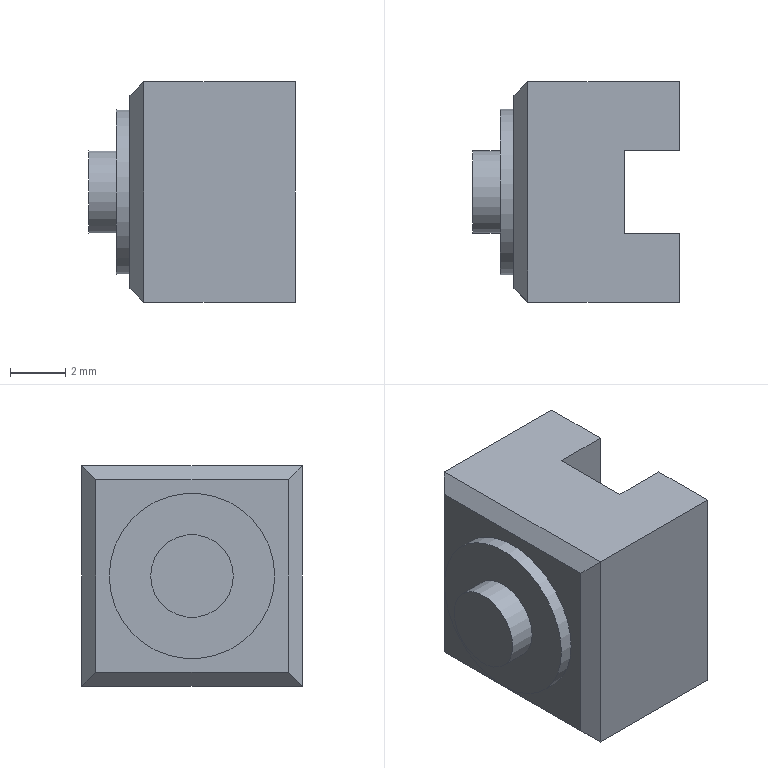Component | NX | IR_THERMAL_IMAGER | 1 solid | 18 faces | box 7.5 x 8 x 8 mm | volume 353 mm3 | plane 16 | cylinder 2 | commonest cylinder face diameters 6 x1 3 x1
STEP:
#1=CARTESIAN_POINT('',(0.,0.,0.));
#2=DIRECTION('',(0.,0.,1.));
#3=DIRECTION('',(1.,0.,0.));
#4=AXIS2_PLACEMENT_3D('',#1,#2,#3);
#5=CARTESIAN_POINT('',(-16.5,4.,12.5));
#6=VERTEX_POINT('',#5);
#7=CARTESIAN_POINT('',(-11.,4.,12.5));
#8=VERTEX_POINT('',#7);
#9=CARTESIAN_POINT('',(-17.,4.,12.5));
#10=DIRECTION('',(1.,0.,0.));
#11=VECTOR('',#10,1.);
#12=LINE('',#9,#11);
#13=CARTESIAN_POINT('',(-17.,4.,12.5));
#14=DIRECTION('',(0.,0.,1.));
#15=DIRECTION('',(0.,1.,-0.));
#16=AXIS2_PLACEMENT_3D('',#13,#14,#15);
#17=PLANE('',#16);
#18=CARTESIAN_POINT('',(0.,0.));
#19=DIRECTION('',(0.,-1.));
#20=VECTOR('',#19,1.);
#21=LINE('',#18,#20);
#22=(GEOMETRIC_REPRESENTATION_CONTEXT(2)PARAMETRIC_REPRESENTATION_CONTEXT()REPRESENTATION_CONTEXT('',''));
#23=DEFINITIONAL_REPRESENTATION('',(#21),#22);
#24=PCURVE('',#17,#23);
#25=CARTESIAN_POINT('',(-17.,4.,4.5));
#26=DIRECTION('',(0.,1.,-0.));
#27=DIRECTION('',(0.,-0.,-1.));
#28=AXIS2_PLACEMENT_3D('',#25,#26,#27);
#29=PLANE('',#28);
#30=CARTESIAN_POINT('',(-8.,0.));
#31=DIRECTION('',(0.,-1.));
#32=VECTOR('',#31,1.);
#33=LINE('',#30,#32);
#34=(GEOMETRIC_REPRESENTATION_CONTEXT(2)PARAMETRIC_REPRESENTATION_CONTEXT()REPRESENTATION_CONTEXT('',''));
#35=DEFINITIONAL_REPRESENTATION('',(#33),#34);
#36=PCURVE('',#29,#35);
#37=SURFACE_CURVE('',#12,(#24,#36),.PCURVE_S1.);
#38=EDGE_CURVE('',#6,#8,#37,.T.);
#39=ORIENTED_EDGE('',*,*,#38,.F.);
#40=CARTESIAN_POINT('',(-16.5,-4.,12.5));
#41=VERTEX_POINT('',#40);
#42=CARTESIAN_POINT('',(-16.5,-4.,12.5));
#43=DIRECTION('',(0.,-1.,0.));
#44=VECTOR('',#43,1.);
#45=LINE('',#42,#44);
#46=CARTESIAN_POINT('',(-8.,-0.5));
#47=DIRECTION('',(-1.,0.));
#48=VECTOR('',#47,1.);
#49=LINE('',#46,#48);
#50=(GEOMETRIC_REPRESENTATION_CONTEXT(2)PARAMETRIC_REPRESENTATION_CONTEXT()REPRESENTATION_CONTEXT('',''));
#51=DEFINITIONAL_REPRESENTATION('',(#49),#50);
#52=PCURVE('',#17,#51);
#53=CARTESIAN_POINT('',(-16.5,4.,12.5));
#54=DIRECTION('',(-0.7071,0.,0.7071));
#55=DIRECTION('',(-0.,1.,-0.));
#56=AXIS2_PLACEMENT_3D('',#53,#54,#55);
#57=PLANE('',#56);
#58=CARTESIAN_POINT('',(-8.,0.));
#59=DIRECTION('',(-1.,0.));
#60=VECTOR('',#59,1.);
#61=LINE('',#58,#60);
#62=(GEOMETRIC_REPRESENTATION_CONTEXT(2)PARAMETRIC_REPRESENTATION_CONTEXT()REPRESENTATION_CONTEXT('',''));
#63=DEFINITIONAL_REPRESENTATION('',(#61),#62);
#64=PCURVE('',#57,#63);
#65=SURFACE_CURVE('',#45,(#52,#64),.PCURVE_S1.);
#66=EDGE_CURVE('',#6,#41,#65,.T.);
#67=ORIENTED_EDGE('',*,*,#66,.T.);
#68=CARTESIAN_POINT('',(-11.,-4.,12.5));
#69=VERTEX_POINT('',#68);
#70=CARTESIAN_POINT('',(-17.,-4.,12.5));
#71=DIRECTION('',(1.,0.,0.));
#72=VECTOR('',#71,1.);
#73=LINE('',#70,#72);
#74=CARTESIAN_POINT('',(-8.,0.));
#75=DIRECTION('',(0.,-1.));
#76=VECTOR('',#75,1.);
#77=LINE('',#74,#76);
#78=(GEOMETRIC_REPRESENTATION_CONTEXT(2)PARAMETRIC_REPRESENTATION_CONTEXT()REPRESENTATION_CONTEXT('',''));
#79=DEFINITIONAL_REPRESENTATION('',(#77),#78);
#80=PCURVE('',#17,#79);
#81=CARTESIAN_POINT('',(-17.,-4.,12.5));
#82=DIRECTION('',(0.,-1.,0.));
#83=DIRECTION('',(0.,0.,1.));
#84=AXIS2_PLACEMENT_3D('',#81,#82,#83);
#85=PLANE('',#84);
#86=CARTESIAN_POINT('',(0.,0.));
#87=DIRECTION('',(0.,-1.));
#88=VECTOR('',#87,1.);
#89=LINE('',#86,#88);
#90=(GEOMETRIC_REPRESENTATION_CONTEXT(2)PARAMETRIC_REPRESENTATION_CONTEXT()REPRESENTATION_CONTEXT('',''));
#91=DEFINITIONAL_REPRESENTATION('',(#89),#90);
#92=PCURVE('',#85,#91);
#93=SURFACE_CURVE('',#73,(#80,#92),.PCURVE_S1.);
#94=EDGE_CURVE('',#41,#69,#93,.T.);
#95=ORIENTED_EDGE('',*,*,#94,.T.);
#96=CARTESIAN_POINT('',(-11.,-1.5,12.5));
#97=VERTEX_POINT('',#96);
#98=CARTESIAN_POINT('',(-11.,4.,12.5));
#99=DIRECTION('',(0.,-1.,0.));
#100=VECTOR('',#99,1.);
#101=LINE('',#98,#100);
#102=CARTESIAN_POINT('',(0.,-6.));
#103=DIRECTION('',(-1.,0.));
#104=VECTOR('',#103,1.);
#105=LINE('',#102,#104);
#106=(GEOMETRIC_REPRESENTATION_CONTEXT(2)PARAMETRIC_REPRESENTATION_CONTEXT()REPRESENTATION_CONTEXT('',''));
#107=DEFINITIONAL_REPRESENTATION('',(#105),#106);
#108=PCURVE('',#17,#107);
#109=CARTESIAN_POINT('',(-11.,0.,8.5));
#110=DIRECTION('',(1.,0.,0.));
#111=DIRECTION('',(0.,0.,-1.));
#112=AXIS2_PLACEMENT_3D('',#109,#110,#111);
#113=PLANE('',#112);
#114=CARTESIAN_POINT('',(-4.,4.));
#115=DIRECTION('',(-0.,-1.));
#116=VECTOR('',#115,1.);
#117=LINE('',#114,#116);
#118=(GEOMETRIC_REPRESENTATION_CONTEXT(2)PARAMETRIC_REPRESENTATION_CONTEXT()REPRESENTATION_CONTEXT('',''));
#119=DEFINITIONAL_REPRESENTATION('',(#117),#118);
#120=PCURVE('',#113,#119);
#121=SURFACE_CURVE('',#101,(#108,#120),.PCURVE_S1.);
#122=EDGE_CURVE('',#97,#69,#121,.T.);
#123=ORIENTED_EDGE('',*,*,#122,.F.);
#124=CARTESIAN_POINT('',(-13.,-1.5,12.5));
#125=VERTEX_POINT('',#124);
#126=CARTESIAN_POINT('',(-11.,-1.5,12.5));
#127=DIRECTION('',(-1.,0.,0.));
#128=VECTOR('',#127,1.);
#129=LINE('',#126,#128);
#130=CARTESIAN_POINT('',(-5.5,-6.));
#131=DIRECTION('',(0.,1.));
#132=VECTOR('',#131,1.);
#133=LINE('',#130,#132);
#134=(GEOMETRIC_REPRESENTATION_CONTEXT(2)PARAMETRIC_REPRESENTATION_CONTEXT()REPRESENTATION_CONTEXT('',''));
#135=DEFINITIONAL_REPRESENTATION('',(#133),#134);
#136=PCURVE('',#17,#135);
#137=CARTESIAN_POINT('',(-11.,-1.5,13.3));
#138=DIRECTION('',(0.,-1.,0.));
#139=DIRECTION('',(0.,0.,1.));
#140=AXIS2_PLACEMENT_3D('',#137,#138,#139);
#141=PLANE('',#140);
#142=CARTESIAN_POINT('',(-0.8,0.));
#143=DIRECTION('',(0.,1.));
#144=VECTOR('',#143,1.);
#145=LINE('',#142,#144);
#146=(GEOMETRIC_REPRESENTATION_CONTEXT(2)PARAMETRIC_REPRESENTATION_CONTEXT()REPRESENTATION_CONTEXT('',''));
#147=DEFINITIONAL_REPRESENTATION('',(#145),#146);
#148=PCURVE('',#141,#147);
#149=SURFACE_CURVE('',#129,(#136,#148),.PCURVE_S1.);
#150=EDGE_CURVE('',#97,#125,#149,.T.);
#151=ORIENTED_EDGE('',*,*,#150,.T.);
#152=CARTESIAN_POINT('',(-13.,1.5,12.5));
#153=VERTEX_POINT('',#152);
#154=CARTESIAN_POINT('',(-13.,-1.5,12.5));
#155=DIRECTION('',(0.,1.,-0.));
#156=VECTOR('',#155,1.);
#157=LINE('',#154,#156);
#158=CARTESIAN_POINT('',(-5.5,-4.));
#159=DIRECTION('',(1.,0.));
#160=VECTOR('',#159,1.);
#161=LINE('',#158,#160);
#162=(GEOMETRIC_REPRESENTATION_CONTEXT(2)PARAMETRIC_REPRESENTATION_CONTEXT()REPRESENTATION_CONTEXT('',''));
#163=DEFINITIONAL_REPRESENTATION('',(#161),#162);
#164=PCURVE('',#17,#163);
#165=CARTESIAN_POINT('',(-13.,-1.5,13.3));
#166=DIRECTION('',(-1.,0.,0.));
#167=DIRECTION('',(0.,0.,1.));
#168=AXIS2_PLACEMENT_3D('',#165,#166,#167);
#169=PLANE('',#168);
#170=CARTESIAN_POINT('',(-0.8,0.));
#171=DIRECTION('',(-0.,1.));
#172=VECTOR('',#171,1.);
#173=LINE('',#170,#172);
#174=(GEOMETRIC_REPRESENTATION_CONTEXT(2)PARAMETRIC_REPRESENTATION_CONTEXT()REPRESENTATION_CONTEXT('',''));
#175=DEFINITIONAL_REPRESENTATION('',(#173),#174);
#176=PCURVE('',#169,#175);
#177=SURFACE_CURVE('',#157,(#164,#176),.PCURVE_S1.);
#178=EDGE_CURVE('',#125,#153,#177,.T.);
#179=ORIENTED_EDGE('',*,*,#178,.T.);
#180=CARTESIAN_POINT('',(-11.,1.5,12.5));
#181=VERTEX_POINT('',#180);
#182=CARTESIAN_POINT('',(-13.,1.5,12.5));
#183=DIRECTION('',(1.,0.,0.));
#184=VECTOR('',#183,1.);
#185=LINE('',#182,#184);
#186=CARTESIAN_POINT('',(-2.5,-4.));
#187=DIRECTION('',(0.,-1.));
#188=VECTOR('',#187,1.);
#189=LINE('',#186,#188);
#190=(GEOMETRIC_REPRESENTATION_CONTEXT(2)PARAMETRIC_REPRESENTATION_CONTEXT()REPRESENTATION_CONTEXT('',''));
#191=DEFINITIONAL_REPRESENTATION('',(#189),#190);
#192=PCURVE('',#17,#191);
#193=CARTESIAN_POINT('',(-13.,1.5,13.3));
#194=DIRECTION('',(0.,1.,0.));
#195=DIRECTION('',(0.,0.,-1.));
#196=AXIS2_PLACEMENT_3D('',#193,#194,#195);
#197=PLANE('',#196);
#198=CARTESIAN_POINT('',(0.8,0.));
#199=DIRECTION('',(0.,-1.));
#200=VECTOR('',#199,1.);
#201=LINE('',#198,#200);
#202=(GEOMETRIC_REPRESENTATION_CONTEXT(2)PARAMETRIC_REPRESENTATION_CONTEXT()REPRESENTATION_CONTEXT('',''));
#203=DEFINITIONAL_REPRESENTATION('',(#201),#202);
#204=PCURVE('',#197,#203);
#205=SURFACE_CURVE('',#185,(#192,#204),.PCURVE_S1.);
#206=EDGE_CURVE('',#153,#181,#205,.T.);
#207=ORIENTED_EDGE('',*,*,#206,.T.);
#208=CARTESIAN_POINT('',(-11.,4.,12.5));
#209=DIRECTION('',(0.,-1.,0.));
#210=VECTOR('',#209,1.);
#211=LINE('',#208,#210);
#212=CARTESIAN_POINT('',(0.,-6.));
#213=DIRECTION('',(-1.,0.));
#214=VECTOR('',#213,1.);
#215=LINE('',#212,#214);
#216=(GEOMETRIC_REPRESENTATION_CONTEXT(2)PARAMETRIC_REPRESENTATION_CONTEXT()REPRESENTATION_CONTEXT('',''));
#217=DEFINITIONAL_REPRESENTATION('',(#215),#216);
#218=PCURVE('',#17,#217);
#219=CARTESIAN_POINT('',(-11.,0.,8.5));
#220=DIRECTION('',(1.,0.,0.));
#221=DIRECTION('',(0.,0.,-1.));
#222=AXIS2_PLACEMENT_3D('',#219,#220,#221);
#223=PLANE('',#222);
#224=CARTESIAN_POINT('',(-4.,4.));
#225=DIRECTION('',(-0.,-1.));
#226=VECTOR('',#225,1.);
#227=LINE('',#224,#226);
#228=(GEOMETRIC_REPRESENTATION_CONTEXT(2)PARAMETRIC_REPRESENTATION_CONTEXT()REPRESENTATION_CONTEXT('',''));
#229=DEFINITIONAL_REPRESENTATION('',(#227),#228);
#230=PCURVE('',#223,#229);
#231=SURFACE_CURVE('',#211,(#218,#230),.PCURVE_S1.);
#232=EDGE_CURVE('',#8,#181,#231,.T.);
#233=ORIENTED_EDGE('',*,*,#232,.F.);
#234=EDGE_LOOP('',(#39,#67,#95,#123,#151,#179,#207,#233));
#235=FACE_BOUND('',#234,.T.);
#236=ADVANCED_FACE('',(#235),#17,.T.);
#237=ORIENTED_EDGE('',*,*,#232,.T.);
#238=CARTESIAN_POINT('',(-11.,1.5,4.5));
#239=VERTEX_POINT('',#238);
#240=CARTESIAN_POINT('',(-11.,1.5,13.3));
#241=DIRECTION('',(0.,0.,-1.));
#242=VECTOR('',#241,1.);
#243=LINE('',#240,#242);
#244=CARTESIAN_POINT('',(-4.8,1.5));
#245=DIRECTION('',(1.,0.));
#246=VECTOR('',#245,1.);
#247=LINE('',#244,#246);
#248=(GEOMETRIC_REPRESENTATION_CONTEXT(2)PARAMETRIC_REPRESENTATION_CONTEXT()REPRESENTATION_CONTEXT('',''));
#249=DEFINITIONAL_REPRESENTATION('',(#247),#248);
#250=PCURVE('',#223,#249);
#251=CARTESIAN_POINT('',(0.,-2.));
#252=DIRECTION('',(1.,0.));
#253=VECTOR('',#252,1.);
#254=LINE('',#251,#253);
#255=(GEOMETRIC_REPRESENTATION_CONTEXT(2)PARAMETRIC_REPRESENTATION_CONTEXT()REPRESENTATION_CONTEXT('',''));
#256=DEFINITIONAL_REPRESENTATION('',(#254),#255);
#257=PCURVE('',#197,#256);
#258=SURFACE_CURVE('',#243,(#250,#257),.PCURVE_S1.);
#259=EDGE_CURVE('',#181,#239,#258,.T.);
#260=ORIENTED_EDGE('',*,*,#259,.T.);
#261=CARTESIAN_POINT('',(-11.,4.,4.5));
#262=VERTEX_POINT('',#261);
#263=CARTESIAN_POINT('',(-11.,-4.,4.5));
#264=DIRECTION('',(0.,1.,-0.));
#265=VECTOR('',#264,1.);
#266=LINE('',#263,#265);
#267=CARTESIAN_POINT('',(4.,-4.));
#268=DIRECTION('',(0.,1.));
#269=VECTOR('',#268,1.);
#270=LINE('',#267,#269);
#271=(GEOMETRIC_REPRESENTATION_CONTEXT(2)PARAMETRIC_REPRESENTATION_CONTEXT()REPRESENTATION_CONTEXT('',''));
#272=DEFINITIONAL_REPRESENTATION('',(#270),#271);
#273=PCURVE('',#223,#272);
#274=CARTESIAN_POINT('',(-17.,-4.,4.5));
#275=DIRECTION('',(0.,-0.,-1.));
#276=DIRECTION('',(0.,-1.,0.));
#277=AXIS2_PLACEMENT_3D('',#274,#275,#276);
#278=PLANE('',#277);
#279=CARTESIAN_POINT('',(0.,-6.));
#280=DIRECTION('',(-1.,0.));
#281=VECTOR('',#280,1.);
#282=LINE('',#279,#281);
#283=(GEOMETRIC_REPRESENTATION_CONTEXT(2)PARAMETRIC_REPRESENTATION_CONTEXT()REPRESENTATION_CONTEXT('',''));
#284=DEFINITIONAL_REPRESENTATION('',(#282),#283);
#285=PCURVE('',#278,#284);
#286=SURFACE_CURVE('',#266,(#273,#285),.PCURVE_S1.);
#287=EDGE_CURVE('',#239,#262,#286,.T.);
#288=ORIENTED_EDGE('',*,*,#287,.T.);
#289=CARTESIAN_POINT('',(-11.,4.,4.5));
#290=DIRECTION('',(0.,0.,1.));
#291=VECTOR('',#290,1.);
#292=LINE('',#289,#291);
#293=CARTESIAN_POINT('',(4.,4.));
#294=DIRECTION('',(-1.,0.));
#295=VECTOR('',#294,1.);
#296=LINE('',#293,#295);
#297=(GEOMETRIC_REPRESENTATION_CONTEXT(2)PARAMETRIC_REPRESENTATION_CONTEXT()REPRESENTATION_CONTEXT('',''));
#298=DEFINITIONAL_REPRESENTATION('',(#296),#297);
#299=PCURVE('',#223,#298);
#300=CARTESIAN_POINT('',(0.,-6.));
#301=DIRECTION('',(-1.,0.));
#302=VECTOR('',#301,1.);
#303=LINE('',#300,#302);
#304=(GEOMETRIC_REPRESENTATION_CONTEXT(2)PARAMETRIC_REPRESENTATION_CONTEXT()REPRESENTATION_CONTEXT('',''));
#305=DEFINITIONAL_REPRESENTATION('',(#303),#304);
#306=PCURVE('',#29,#305);
#307=SURFACE_CURVE('',#292,(#299,#306),.PCURVE_S1.);
#308=EDGE_CURVE('',#262,#8,#307,.T.);
#309=ORIENTED_EDGE('',*,*,#308,.T.);
#310=EDGE_LOOP('',(#237,#260,#288,#309));
#311=FACE_BOUND('',#310,.T.);
#312=ADVANCED_FACE('',(#311),#223,.T.);
#313=ORIENTED_EDGE('',*,*,#94,.F.);
#314=CARTESIAN_POINT('',(-16.5,-4.,4.5));
#315=VERTEX_POINT('',#314);
#316=CARTESIAN_POINT('',(-16.5,-4.,4.5));
#317=DIRECTION('',(0.,-0.,-1.));
#318=VECTOR('',#317,1.);
#319=LINE('',#316,#318);
#320=CARTESIAN_POINT('',(-8.,-0.5));
#321=DIRECTION('',(-1.,0.));
#322=VECTOR('',#321,1.);
#323=LINE('',#320,#322);
#324=(GEOMETRIC_REPRESENTATION_CONTEXT(2)PARAMETRIC_REPRESENTATION_CONTEXT()REPRESENTATION_CONTEXT('',''));
#325=DEFINITIONAL_REPRESENTATION('',(#323),#324);
#326=PCURVE('',#85,#325);
#327=CARTESIAN_POINT('',(-16.5,-4.,12.5));
#328=DIRECTION('',(-0.7071,-0.7071,0.));
#329=DIRECTION('',(0.,0.,1.));
#330=AXIS2_PLACEMENT_3D('',#327,#328,#329);
#331=PLANE('',#330);
#332=CARTESIAN_POINT('',(-8.,0.));
#333=DIRECTION('',(-1.,0.));
#334=VECTOR('',#333,1.);
#335=LINE('',#332,#334);
#336=(GEOMETRIC_REPRESENTATION_CONTEXT(2)PARAMETRIC_REPRESENTATION_CONTEXT()REPRESENTATION_CONTEXT('',''));
#337=DEFINITIONAL_REPRESENTATION('',(#335),#336);
#338=PCURVE('',#331,#337);
#339=SURFACE_CURVE('',#319,(#326,#338),.PCURVE_S1.);
#340=EDGE_CURVE('',#41,#315,#339,.T.);
#341=ORIENTED_EDGE('',*,*,#340,.T.);
#342=CARTESIAN_POINT('',(-11.,-4.,4.5));
#343=VERTEX_POINT('',#342);
#344=CARTESIAN_POINT('',(-17.,-4.,4.5));
#345=DIRECTION('',(1.,0.,0.));
#346=VECTOR('',#345,1.);
#347=LINE('',#344,#346);
#348=CARTESIAN_POINT('',(-8.,0.));
#349=DIRECTION('',(0.,-1.));
#350=VECTOR('',#349,1.);
#351=LINE('',#348,#350);
#352=(GEOMETRIC_REPRESENTATION_CONTEXT(2)PARAMETRIC_REPRESENTATION_CONTEXT()REPRESENTATION_CONTEXT('',''));
#353=DEFINITIONAL_REPRESENTATION('',(#351),#352);
#354=PCURVE('',#85,#353);
#355=CARTESIAN_POINT('',(0.,0.));
#356=DIRECTION('',(0.,-1.));
#357=VECTOR('',#356,1.);
#358=LINE('',#355,#357);
#359=(GEOMETRIC_REPRESENTATION_CONTEXT(2)PARAMETRIC_REPRESENTATION_CONTEXT()REPRESENTATION_CONTEXT('',''));
#360=DEFINITIONAL_REPRESENTATION('',(#358),#359);
#361=PCURVE('',#278,#360);
#362=SURFACE_CURVE('',#347,(#354,#361),.PCURVE_S1.);
#363=EDGE_CURVE('',#315,#343,#362,.T.);
#364=ORIENTED_EDGE('',*,*,#363,.T.);
#365=CARTESIAN_POINT('',(-11.,-4.,12.5));
#366=DIRECTION('',(0.,-0.,-1.));
#367=VECTOR('',#366,1.);
#368=LINE('',#365,#367);
#369=CARTESIAN_POINT('',(0.,-6.));
#370=DIRECTION('',(-1.,0.));
#371=VECTOR('',#370,1.);
#372=LINE('',#369,#371);
#373=(GEOMETRIC_REPRESENTATION_CONTEXT(2)PARAMETRIC_REPRESENTATION_CONTEXT()REPRESENTATION_CONTEXT('',''));
#374=DEFINITIONAL_REPRESENTATION('',(#372),#373);
#375=PCURVE('',#85,#374);
#376=CARTESIAN_POINT('',(-4.,-4.));
#377=DIRECTION('',(1.,-0.));
#378=VECTOR('',#377,1.);
#379=LINE('',#376,#378);
#380=(GEOMETRIC_REPRESENTATION_CONTEXT(2)PARAMETRIC_REPRESENTATION_CONTEXT()REPRESENTATION_CONTEXT('',''));
#381=DEFINITIONAL_REPRESENTATION('',(#379),#380);
#382=PCURVE('',#113,#381);
#383=SURFACE_CURVE('',#368,(#375,#382),.PCURVE_S1.);
#384=EDGE_CURVE('',#69,#343,#383,.T.);
#385=ORIENTED_EDGE('',*,*,#384,.F.);
#386=EDGE_LOOP('',(#313,#341,#364,#385));
#387=FACE_BOUND('',#386,.T.);
#388=ADVANCED_FACE('',(#387),#85,.T.);
#389=ORIENTED_EDGE('',*,*,#363,.F.);
#390=CARTESIAN_POINT('',(-16.5,4.,4.5));
#391=VERTEX_POINT('',#390);
#392=CARTESIAN_POINT('',(-16.5,4.,4.5));
#393=DIRECTION('',(0.,1.,-0.));
#394=VECTOR('',#393,1.);
#395=LINE('',#392,#394);
#396=CARTESIAN_POINT('',(-8.,-0.5));
#397=DIRECTION('',(-1.,0.));
#398=VECTOR('',#397,1.);
#399=LINE('',#396,#398);
#400=(GEOMETRIC_REPRESENTATION_CONTEXT(2)PARAMETRIC_REPRESENTATION_CONTEXT()REPRESENTATION_CONTEXT('',''));
#401=DEFINITIONAL_REPRESENTATION('',(#399),#400);
#402=PCURVE('',#278,#401);
#403=CARTESIAN_POINT('',(-16.5,-4.,4.5));
#404=DIRECTION('',(-0.7071,-0.,-0.7071));
#405=DIRECTION('',(0.,-1.,0.));
#406=AXIS2_PLACEMENT_3D('',#403,#404,#405);
#407=PLANE('',#406);
#408=CARTESIAN_POINT('',(-8.,0.));
#409=DIRECTION('',(-1.,-0.));
#410=VECTOR('',#409,1.);
#411=LINE('',#408,#410);
#412=(GEOMETRIC_REPRESENTATION_CONTEXT(2)PARAMETRIC_REPRESENTATION_CONTEXT()REPRESENTATION_CONTEXT('',''));
#413=DEFINITIONAL_REPRESENTATION('',(#411),#412);
#414=PCURVE('',#407,#413);
#415=SURFACE_CURVE('',#395,(#402,#414),.PCURVE_S1.);
#416=EDGE_CURVE('',#315,#391,#415,.T.);
#417=ORIENTED_EDGE('',*,*,#416,.T.);
#418=CARTESIAN_POINT('',(-17.,4.,4.5));
#419=DIRECTION('',(1.,0.,0.));
#420=VECTOR('',#419,1.);
#421=LINE('',#418,#420);
#422=CARTESIAN_POINT('',(-8.,0.));
#423=DIRECTION('',(0.,-1.));
#424=VECTOR('',#423,1.);
#425=LINE('',#422,#424);
#426=(GEOMETRIC_REPRESENTATION_CONTEXT(2)PARAMETRIC_REPRESENTATION_CONTEXT()REPRESENTATION_CONTEXT('',''));
#427=DEFINITIONAL_REPRESENTATION('',(#425),#426);
#428=PCURVE('',#278,#427);
#429=CARTESIAN_POINT('',(0.,0.));
#430=DIRECTION('',(0.,-1.));
#431=VECTOR('',#430,1.);
#432=LINE('',#429,#431);
#433=(GEOMETRIC_REPRESENTATION_CONTEXT(2)PARAMETRIC_REPRESENTATION_CONTEXT()REPRESENTATION_CONTEXT('',''));
#434=DEFINITIONAL_REPRESENTATION('',(#432),#433);
#435=PCURVE('',#29,#434);
#436=SURFACE_CURVE('',#421,(#428,#435),.PCURVE_S1.);
#437=EDGE_CURVE('',#391,#262,#436,.T.);
#438=ORIENTED_EDGE('',*,*,#437,.T.);
#439=ORIENTED_EDGE('',*,*,#287,.F.);
#440=CARTESIAN_POINT('',(-13.,1.5,4.5));
#441=VERTEX_POINT('',#440);
#442=CARTESIAN_POINT('',(-13.,1.5,4.5));
#443=DIRECTION('',(1.,0.,0.));
#444=VECTOR('',#443,1.);
#445=LINE('',#442,#444);
#446=CARTESIAN_POINT('',(-5.5,-4.));
#447=DIRECTION('',(0.,-1.));
#448=VECTOR('',#447,1.);
#449=LINE('',#446,#448);
#450=(GEOMETRIC_REPRESENTATION_CONTEXT(2)PARAMETRIC_REPRESENTATION_CONTEXT()REPRESENTATION_CONTEXT('',''));
#451=DEFINITIONAL_REPRESENTATION('',(#449),#450);
#452=PCURVE('',#278,#451);
#453=CARTESIAN_POINT('',(8.8,0.));
#454=DIRECTION('',(0.,-1.));
#455=VECTOR('',#454,1.);
#456=LINE('',#453,#455);
#457=(GEOMETRIC_REPRESENTATION_CONTEXT(2)PARAMETRIC_REPRESENTATION_CONTEXT()REPRESENTATION_CONTEXT('',''));
#458=DEFINITIONAL_REPRESENTATION('',(#456),#457);
#459=PCURVE('',#197,#458);
#460=SURFACE_CURVE('',#445,(#452,#459),.PCURVE_S1.);
#461=EDGE_CURVE('',#441,#239,#460,.T.);
#462=ORIENTED_EDGE('',*,*,#461,.F.);
#463=CARTESIAN_POINT('',(-13.,-1.5,4.5));
#464=VERTEX_POINT('',#463);
#465=CARTESIAN_POINT('',(-13.,-1.5,4.5));
#466=DIRECTION('',(0.,1.,0.));
#467=VECTOR('',#466,1.);
#468=LINE('',#465,#467);
#469=CARTESIAN_POINT('',(-2.5,-4.));
#470=DIRECTION('',(-1.,0.));
#471=VECTOR('',#470,1.);
#472=LINE('',#469,#471);
#473=(GEOMETRIC_REPRESENTATION_CONTEXT(2)PARAMETRIC_REPRESENTATION_CONTEXT()REPRESENTATION_CONTEXT('',''));
#474=DEFINITIONAL_REPRESENTATION('',(#472),#473);
#475=PCURVE('',#278,#474);
#476=CARTESIAN_POINT('',(-8.8,0.));
#477=DIRECTION('',(0.,1.));
#478=VECTOR('',#477,1.);
#479=LINE('',#476,#478);
#480=(GEOMETRIC_REPRESENTATION_CONTEXT(2)PARAMETRIC_REPRESENTATION_CONTEXT()REPRESENTATION_CONTEXT('',''));
#481=DEFINITIONAL_REPRESENTATION('',(#479),#480);
#482=PCURVE('',#169,#481);
#483=SURFACE_CURVE('',#468,(#475,#482),.PCURVE_S1.);
#484=EDGE_CURVE('',#464,#441,#483,.T.);
#485=ORIENTED_EDGE('',*,*,#484,.F.);
#486=CARTESIAN_POINT('',(-11.,-1.5,4.5));
#487=VERTEX_POINT('',#486);
#488=CARTESIAN_POINT('',(-11.,-1.5,4.5));
#489=DIRECTION('',(-1.,0.,0.));
#490=VECTOR('',#489,1.);
#491=LINE('',#488,#490);
#492=CARTESIAN_POINT('',(-2.5,-6.));
#493=DIRECTION('',(0.,1.));
#494=VECTOR('',#493,1.);
#495=LINE('',#492,#494);
#496=(GEOMETRIC_REPRESENTATION_CONTEXT(2)PARAMETRIC_REPRESENTATION_CONTEXT()REPRESENTATION_CONTEXT('',''));
#497=DEFINITIONAL_REPRESENTATION('',(#495),#496);
#498=PCURVE('',#278,#497);
#499=CARTESIAN_POINT('',(-8.8,0.));
#500=DIRECTION('',(0.,1.));
#501=VECTOR('',#500,1.);
#502=LINE('',#499,#501);
#503=(GEOMETRIC_REPRESENTATION_CONTEXT(2)PARAMETRIC_REPRESENTATION_CONTEXT()REPRESENTATION_CONTEXT('',''));
#504=DEFINITIONAL_REPRESENTATION('',(#502),#503);
#505=PCURVE('',#141,#504);
#506=SURFACE_CURVE('',#491,(#498,#505),.PCURVE_S1.);
#507=EDGE_CURVE('',#487,#464,#506,.T.);
#508=ORIENTED_EDGE('',*,*,#507,.F.);
#509=CARTESIAN_POINT('',(-11.,-4.,4.5));
#510=DIRECTION('',(0.,1.,-0.));
#511=VECTOR('',#510,1.);
#512=LINE('',#509,#511);
#513=CARTESIAN_POINT('',(0.,-6.));
#514=DIRECTION('',(-1.,0.));
#515=VECTOR('',#514,1.);
#516=LINE('',#513,#515);
#517=(GEOMETRIC_REPRESENTATION_CONTEXT(2)PARAMETRIC_REPRESENTATION_CONTEXT()REPRESENTATION_CONTEXT('',''));
#518=DEFINITIONAL_REPRESENTATION('',(#516),#517);
#519=PCURVE('',#278,#518);
#520=CARTESIAN_POINT('',(4.,-4.));
#521=DIRECTION('',(0.,1.));
#522=VECTOR('',#521,1.);
#523=LINE('',#520,#522);
#524=(GEOMETRIC_REPRESENTATION_CONTEXT(2)PARAMETRIC_REPRESENTATION_CONTEXT()REPRESENTATION_CONTEXT('',''));
#525=DEFINITIONAL_REPRESENTATION('',(#523),#524);
#526=PCURVE('',#113,#525);
#527=SURFACE_CURVE('',#512,(#519,#526),.PCURVE_S1.);
#528=EDGE_CURVE('',#343,#487,#527,.T.);
#529=ORIENTED_EDGE('',*,*,#528,.F.);
#530=EDGE_LOOP('',(#389,#417,#438,#439,#462,#485,#508,#529));
#531=FACE_BOUND('',#530,.T.);
#532=ADVANCED_FACE('',(#531),#278,.T.);
#533=ORIENTED_EDGE('',*,*,#437,.F.);
#534=CARTESIAN_POINT('',(-16.5,4.,12.5));
#535=DIRECTION('',(0.,0.,1.));
#536=VECTOR('',#535,1.);
#537=LINE('',#534,#536);
#538=CARTESIAN_POINT('',(-8.,-0.5));
#539=DIRECTION('',(-1.,0.));
#540=VECTOR('',#539,1.);
#541=LINE('',#538,#540);
#542=(GEOMETRIC_REPRESENTATION_CONTEXT(2)PARAMETRIC_REPRESENTATION_CONTEXT()REPRESENTATION_CONTEXT('',''));
#543=DEFINITIONAL_REPRESENTATION('',(#541),#542);
#544=PCURVE('',#29,#543);
#545=CARTESIAN_POINT('',(-16.5,4.,4.5));
#546=DIRECTION('',(-0.7071,0.7071,-0.));
#547=DIRECTION('',(0.,-0.,-1.));
#548=AXIS2_PLACEMENT_3D('',#545,#546,#547);
#549=PLANE('',#548);
#550=CARTESIAN_POINT('',(-8.,0.));
#551=DIRECTION('',(-1.,0.));
#552=VECTOR('',#551,1.);
#553=LINE('',#550,#552);
#554=(GEOMETRIC_REPRESENTATION_CONTEXT(2)PARAMETRIC_REPRESENTATION_CONTEXT()REPRESENTATION_CONTEXT('',''));
#555=DEFINITIONAL_REPRESENTATION('',(#553),#554);
#556=PCURVE('',#549,#555);
#557=SURFACE_CURVE('',#537,(#544,#556),.PCURVE_S1.);
#558=EDGE_CURVE('',#391,#6,#557,.T.);
#559=ORIENTED_EDGE('',*,*,#558,.T.);
#560=ORIENTED_EDGE('',*,*,#38,.T.);
#561=ORIENTED_EDGE('',*,*,#308,.F.);
#562=EDGE_LOOP('',(#533,#559,#560,#561));
#563=FACE_BOUND('',#562,.T.);
#564=ADVANCED_FACE('',(#563),#29,.T.);
#565=CARTESIAN_POINT('',(-17.,-3.5,5.));
#566=VERTEX_POINT('',#565);
#567=CARTESIAN_POINT('',(-17.,-3.5,12.));
#568=VERTEX_POINT('',#567);
#569=CARTESIAN_POINT('',(-17.,-3.5,12.5));
#570=DIRECTION('',(0.,0.,1.));
#571=VECTOR('',#570,1.);
#572=LINE('',#569,#571);
#573=CARTESIAN_POINT('',(-17.,0.,8.5));
#574=DIRECTION('',(1.,0.,0.));
#575=DIRECTION('',(0.,0.,-1.));
#576=AXIS2_PLACEMENT_3D('',#573,#574,#575);
#577=PLANE('',#576);
#578=CARTESIAN_POINT('',(-4.,-3.5));
#579=DIRECTION('',(-1.,0.));
#580=VECTOR('',#579,1.);
#581=LINE('',#578,#580);
#582=(GEOMETRIC_REPRESENTATION_CONTEXT(2)PARAMETRIC_REPRESENTATION_CONTEXT()REPRESENTATION_CONTEXT('',''));
#583=DEFINITIONAL_REPRESENTATION('',(#581),#582);
#584=PCURVE('',#577,#583);
#585=CARTESIAN_POINT('',(0.,0.7071));
#586=DIRECTION('',(1.,0.));
#587=VECTOR('',#586,1.);
#588=LINE('',#585,#587);
#589=(GEOMETRIC_REPRESENTATION_CONTEXT(2)PARAMETRIC_REPRESENTATION_CONTEXT()REPRESENTATION_CONTEXT('',''));
#590=DEFINITIONAL_REPRESENTATION('',(#588),#589);
#591=PCURVE('',#331,#590);
#592=SURFACE_CURVE('',#572,(#584,#591),.PCURVE_S1.);
#593=EDGE_CURVE('',#566,#568,#592,.T.);
#594=ORIENTED_EDGE('',*,*,#593,.T.);
#595=CARTESIAN_POINT('',(-17.,3.5,12.));
#596=VERTEX_POINT('',#595);
#597=CARTESIAN_POINT('',(-17.,4.,12.));
#598=DIRECTION('',(0.,1.,-0.));
#599=VECTOR('',#598,1.);
#600=LINE('',#597,#599);
#601=CARTESIAN_POINT('',(-3.5,4.));
#602=DIRECTION('',(0.,1.));
#603=VECTOR('',#602,1.);
#604=LINE('',#601,#603);
#605=(GEOMETRIC_REPRESENTATION_CONTEXT(2)PARAMETRIC_REPRESENTATION_CONTEXT()REPRESENTATION_CONTEXT('',''));
#606=DEFINITIONAL_REPRESENTATION('',(#604),#605);
#607=PCURVE('',#577,#606);
#608=CARTESIAN_POINT('',(0.,0.7071));
#609=DIRECTION('',(1.,-0.));
#610=VECTOR('',#609,1.);
#611=LINE('',#608,#610);
#612=(GEOMETRIC_REPRESENTATION_CONTEXT(2)PARAMETRIC_REPRESENTATION_CONTEXT()REPRESENTATION_CONTEXT('',''));
#613=DEFINITIONAL_REPRESENTATION('',(#611),#612);
#614=PCURVE('',#57,#613);
#615=SURFACE_CURVE('',#600,(#607,#614),.PCURVE_S1.);
#616=EDGE_CURVE('',#568,#596,#615,.T.);
#617=ORIENTED_EDGE('',*,*,#616,.T.);
#618=CARTESIAN_POINT('',(-17.,3.5,5.));
#619=VERTEX_POINT('',#618);
#620=CARTESIAN_POINT('',(-17.,3.5,4.5));
#621=DIRECTION('',(0.,-0.,-1.));
#622=VECTOR('',#621,1.);
#623=LINE('',#620,#622);
#624=CARTESIAN_POINT('',(4.,3.5));
#625=DIRECTION('',(1.,-0.));
#626=VECTOR('',#625,1.);
#627=LINE('',#624,#626);
#628=(GEOMETRIC_REPRESENTATION_CONTEXT(2)PARAMETRIC_REPRESENTATION_CONTEXT()REPRESENTATION_CONTEXT('',''));
#629=DEFINITIONAL_REPRESENTATION('',(#627),#628);
#630=PCURVE('',#577,#629);
#631=CARTESIAN_POINT('',(0.,0.7071));
#632=DIRECTION('',(1.,0.));
#633=VECTOR('',#632,1.);
#634=LINE('',#631,#633);
#635=(GEOMETRIC_REPRESENTATION_CONTEXT(2)PARAMETRIC_REPRESENTATION_CONTEXT()REPRESENTATION_CONTEXT('',''));
#636=DEFINITIONAL_REPRESENTATION('',(#634),#635);
#637=PCURVE('',#549,#636);
#638=SURFACE_CURVE('',#623,(#630,#637),.PCURVE_S1.);
#639=EDGE_CURVE('',#596,#619,#638,.T.);
#640=ORIENTED_EDGE('',*,*,#639,.T.);
#641=CARTESIAN_POINT('',(-17.,-4.,5.));
#642=DIRECTION('',(0.,-1.,0.));
#643=VECTOR('',#642,1.);
#644=LINE('',#641,#643);
#645=CARTESIAN_POINT('',(3.5,-4.));
#646=DIRECTION('',(-0.,-1.));
#647=VECTOR('',#646,1.);
#648=LINE('',#645,#647);
#649=(GEOMETRIC_REPRESENTATION_CONTEXT(2)PARAMETRIC_REPRESENTATION_CONTEXT()REPRESENTATION_CONTEXT('',''));
#650=DEFINITIONAL_REPRESENTATION('',(#648),#649);
#651=PCURVE('',#577,#650);
#652=CARTESIAN_POINT('',(0.,0.7071));
#653=DIRECTION('',(1.,0.));
#654=VECTOR('',#653,1.);
#655=LINE('',#652,#654);
#656=(GEOMETRIC_REPRESENTATION_CONTEXT(2)PARAMETRIC_REPRESENTATION_CONTEXT()REPRESENTATION_CONTEXT('',''));
#657=DEFINITIONAL_REPRESENTATION('',(#655),#656);
#658=PCURVE('',#407,#657);
#659=SURFACE_CURVE('',#644,(#651,#658),.PCURVE_S1.);
#660=EDGE_CURVE('',#619,#566,#659,.T.);
#661=ORIENTED_EDGE('',*,*,#660,.T.);
#662=EDGE_LOOP('',(#594,#617,#640,#661));
#663=FACE_BOUND('',#662,.T.);
#664=CARTESIAN_POINT('',(-17.,3.,8.5));
#665=VERTEX_POINT('',#664);
#666=CARTESIAN_POINT('',(-17.,0.,8.5));
#667=DIRECTION('',(1.,0.,0.));
#668=DIRECTION('',(0.,1.,0.));
#669=AXIS2_PLACEMENT_3D('',#666,#667,#668);
#670=CIRCLE('',#669,3.);
#671=CARTESIAN_POINT('',(0.,0.));
#672=DIRECTION('',(0.,1.));
#673=AXIS2_PLACEMENT_2D('',#671,#672);
#674=CIRCLE('',#673,3.);
#675=(GEOMETRIC_REPRESENTATION_CONTEXT(2)PARAMETRIC_REPRESENTATION_CONTEXT()REPRESENTATION_CONTEXT('',''));
#676=DEFINITIONAL_REPRESENTATION('',(#674),#675);
#677=PCURVE('',#577,#676);
#678=CARTESIAN_POINT('',(-17.5,0.,8.5));
#679=DIRECTION('',(1.,0.,0.));
#680=DIRECTION('',(0.,0.,-1.));
#681=AXIS2_PLACEMENT_3D('',#678,#679,#680);
#682=CYLINDRICAL_SURFACE('',#681,3.);
#683=CARTESIAN_POINT('',(1.571,0.5));
#684=DIRECTION('',(1.,0.));
#685=VECTOR('',#684,1.);
#686=LINE('',#683,#685);
#687=(GEOMETRIC_REPRESENTATION_CONTEXT(2)PARAMETRIC_REPRESENTATION_CONTEXT()REPRESENTATION_CONTEXT('',''));
#688=DEFINITIONAL_REPRESENTATION('',(#686),#687);
#689=PCURVE('',#682,#688);
#690=SURFACE_CURVE('',#670,(#677,#689),.PCURVE_S1.);
#691=EDGE_CURVE('',#665,#665,#690,.T.);
#692=ORIENTED_EDGE('',*,*,#691,.T.);
#693=EDGE_LOOP('',(#692));
#694=FACE_BOUND('',#693,.T.);
#695=ADVANCED_FACE('',(#663,#694),#577,.F.);
#696=CARTESIAN_POINT('',(-11.,-1.5,13.3));
#697=DIRECTION('',(0.,0.,-1.));
#698=VECTOR('',#697,1.);
#699=LINE('',#696,#698);
#700=CARTESIAN_POINT('',(-4.8,-1.5));
#701=DIRECTION('',(1.,0.));
#702=VECTOR('',#701,1.);
#703=LINE('',#700,#702);
#704=(GEOMETRIC_REPRESENTATION_CONTEXT(2)PARAMETRIC_REPRESENTATION_CONTEXT()REPRESENTATION_CONTEXT('',''));
#705=DEFINITIONAL_REPRESENTATION('',(#703),#704);
#706=PCURVE('',#113,#705);
#707=CARTESIAN_POINT('',(0.,0.));
#708=DIRECTION('',(-1.,0.));
#709=VECTOR('',#708,1.);
#710=LINE('',#707,#709);
#711=(GEOMETRIC_REPRESENTATION_CONTEXT(2)PARAMETRIC_REPRESENTATION_CONTEXT()REPRESENTATION_CONTEXT('',''));
#712=DEFINITIONAL_REPRESENTATION('',(#710),#711);
#713=PCURVE('',#141,#712);
#714=SURFACE_CURVE('',#699,(#706,#713),.PCURVE_S1.);
#715=EDGE_CURVE('',#97,#487,#714,.T.);
#716=ORIENTED_EDGE('',*,*,#715,.F.);
#717=ORIENTED_EDGE('',*,*,#122,.T.);
#718=ORIENTED_EDGE('',*,*,#384,.T.);
#719=ORIENTED_EDGE('',*,*,#528,.T.);
#720=EDGE_LOOP('',(#716,#717,#718,#719));
#721=FACE_BOUND('',#720,.T.);
#722=ADVANCED_FACE('',(#721),#113,.T.);
#723=ORIENTED_EDGE('',*,*,#715,.T.);
#724=ORIENTED_EDGE('',*,*,#507,.T.);
#725=CARTESIAN_POINT('',(-13.,-1.5,13.3));
#726=DIRECTION('',(0.,0.,1.));
#727=VECTOR('',#726,1.);
#728=LINE('',#725,#727);
#729=CARTESIAN_POINT('',(0.,2.));
#730=DIRECTION('',(1.,0.));
#731=VECTOR('',#730,1.);
#732=LINE('',#729,#731);
#733=(GEOMETRIC_REPRESENTATION_CONTEXT(2)PARAMETRIC_REPRESENTATION_CONTEXT()REPRESENTATION_CONTEXT('',''));
#734=DEFINITIONAL_REPRESENTATION('',(#732),#733);
#735=PCURVE('',#141,#734);
#736=CARTESIAN_POINT('',(0.,0.));
#737=DIRECTION('',(1.,0.));
#738=VECTOR('',#737,1.);
#739=LINE('',#736,#738);
#740=(GEOMETRIC_REPRESENTATION_CONTEXT(2)PARAMETRIC_REPRESENTATION_CONTEXT()REPRESENTATION_CONTEXT('',''));
#741=DEFINITIONAL_REPRESENTATION('',(#739),#740);
#742=PCURVE('',#169,#741);
#743=SURFACE_CURVE('',#728,(#735,#742),.PCURVE_S1.);
#744=EDGE_CURVE('',#464,#125,#743,.T.);
#745=ORIENTED_EDGE('',*,*,#744,.T.);
#746=ORIENTED_EDGE('',*,*,#150,.F.);
#747=EDGE_LOOP('',(#723,#724,#745,#746));
#748=FACE_BOUND('',#747,.T.);
#749=ADVANCED_FACE('',(#748),#141,.F.);
#750=ORIENTED_EDGE('',*,*,#744,.F.);
#751=ORIENTED_EDGE('',*,*,#484,.T.);
#752=CARTESIAN_POINT('',(-13.,1.5,13.3));
#753=DIRECTION('',(0.,0.,1.));
#754=VECTOR('',#753,1.);
#755=LINE('',#752,#754);
#756=CARTESIAN_POINT('',(0.,3.));
#757=DIRECTION('',(1.,0.));
#758=VECTOR('',#757,1.);
#759=LINE('',#756,#758);
#760=(GEOMETRIC_REPRESENTATION_CONTEXT(2)PARAMETRIC_REPRESENTATION_CONTEXT()REPRESENTATION_CONTEXT('',''));
#761=DEFINITIONAL_REPRESENTATION('',(#759),#760);
#762=PCURVE('',#169,#761);
#763=CARTESIAN_POINT('',(0.,0.));
#764=DIRECTION('',(-1.,0.));
#765=VECTOR('',#764,1.);
#766=LINE('',#763,#765);
#767=(GEOMETRIC_REPRESENTATION_CONTEXT(2)PARAMETRIC_REPRESENTATION_CONTEXT()REPRESENTATION_CONTEXT('',''));
#768=DEFINITIONAL_REPRESENTATION('',(#766),#767);
#769=PCURVE('',#197,#768);
#770=SURFACE_CURVE('',#755,(#762,#769),.PCURVE_S1.);
#771=EDGE_CURVE('',#441,#153,#770,.T.);
#772=ORIENTED_EDGE('',*,*,#771,.T.);
#773=ORIENTED_EDGE('',*,*,#178,.F.);
#774=EDGE_LOOP('',(#750,#751,#772,#773));
#775=FACE_BOUND('',#774,.T.);
#776=ADVANCED_FACE('',(#775),#169,.F.);
#777=ORIENTED_EDGE('',*,*,#771,.F.);
#778=ORIENTED_EDGE('',*,*,#461,.T.);
#779=ORIENTED_EDGE('',*,*,#259,.F.);
#780=ORIENTED_EDGE('',*,*,#206,.F.);
#781=EDGE_LOOP('',(#777,#778,#779,#780));
#782=FACE_BOUND('',#781,.T.);
#783=ADVANCED_FACE('',(#782),#197,.F.);
#784=CARTESIAN_POINT('',(-17.5,3.,8.5));
#785=VERTEX_POINT('',#784);
#786=CARTESIAN_POINT('',(-17.5,0.,8.5));
#787=DIRECTION('',(1.,0.,0.));
#788=DIRECTION('',(0.,1.,0.));
#789=AXIS2_PLACEMENT_3D('',#786,#787,#788);
#790=CIRCLE('',#789,3.);
#791=CARTESIAN_POINT('',(1.571,0.));
#792=DIRECTION('',(1.,0.));
#793=VECTOR('',#792,1.);
#794=LINE('',#791,#793);
#795=(GEOMETRIC_REPRESENTATION_CONTEXT(2)PARAMETRIC_REPRESENTATION_CONTEXT()REPRESENTATION_CONTEXT('',''));
#796=DEFINITIONAL_REPRESENTATION('',(#794),#795);
#797=PCURVE('',#682,#796);
#798=CARTESIAN_POINT('',(-17.5,0.,8.5));
#799=DIRECTION('',(1.,0.,0.));
#800=DIRECTION('',(0.,0.,-1.));
#801=AXIS2_PLACEMENT_3D('',#798,#799,#800);
#802=PLANE('',#801);
#803=CARTESIAN_POINT('',(0.,0.));
#804=DIRECTION('',(0.,1.));
#805=AXIS2_PLACEMENT_2D('',#803,#804);
#806=CIRCLE('',#805,3.);
#807=(GEOMETRIC_REPRESENTATION_CONTEXT(2)PARAMETRIC_REPRESENTATION_CONTEXT()REPRESENTATION_CONTEXT('',''));
#808=DEFINITIONAL_REPRESENTATION('',(#806),#807);
#809=PCURVE('',#802,#808);
#810=SURFACE_CURVE('',#790,(#797,#809),.PCURVE_S1.);
#811=EDGE_CURVE('',#785,#785,#810,.T.);
#812=ORIENTED_EDGE('',*,*,#811,.T.);
#813=CARTESIAN_POINT('',(-17.5,3.,8.5));
#814=CARTESIAN_POINT('',(-17.,3.,8.5));
#815=B_SPLINE_CURVE_WITH_KNOTS('',1,(#813,#814),.UNSPECIFIED.,.F.,.F.,(2,2),(0.,0.5),.PIECEWISE_BEZIER_KNOTS.);
#816=CARTESIAN_POINT('',(7.854,0.));
#817=DIRECTION('',(0.,1.));
#818=VECTOR('',#817,1.);
#819=LINE('',#816,#818);
#820=(GEOMETRIC_REPRESENTATION_CONTEXT(2)PARAMETRIC_REPRESENTATION_CONTEXT()REPRESENTATION_CONTEXT('',''));
#821=DEFINITIONAL_REPRESENTATION('',(#819),#820);
#822=PCURVE('',#682,#821);
#823=CARTESIAN_POINT('',(1.571,0.));
#824=DIRECTION('',(0.,1.));
#825=VECTOR('',#824,1.);
#826=LINE('',#823,#825);
#827=(GEOMETRIC_REPRESENTATION_CONTEXT(2)PARAMETRIC_REPRESENTATION_CONTEXT()REPRESENTATION_CONTEXT('',''));
#828=DEFINITIONAL_REPRESENTATION('',(#826),#827);
#829=PCURVE('',#682,#828);
#830=SEAM_CURVE('',#815,(#822,#829),.PCURVE_S1.);
#831=EDGE_CURVE('',#785,#665,#830,.T.);
#832=ORIENTED_EDGE('',*,*,#831,.T.);
#833=ORIENTED_EDGE('',*,*,#691,.F.);
#834=ORIENTED_EDGE('',*,*,#831,.F.);
#835=EDGE_LOOP('',(#812,#832,#833,#834));
#836=FACE_BOUND('',#835,.T.);
#837=ADVANCED_FACE('',(#836),#682,.T.);
#838=CARTESIAN_POINT('',(-17.5,1.5,8.5));
#839=VERTEX_POINT('',#838);
#840=CARTESIAN_POINT('',(-17.5,0.,8.5));
#841=DIRECTION('',(-1.,0.,0.));
#842=DIRECTION('',(0.,1.,0.));
#843=AXIS2_PLACEMENT_3D('',#840,#841,#842);
#844=CIRCLE('',#843,1.5);
#845=CARTESIAN_POINT('',(0.,1.5));
#846=CARTESIAN_POINT('',(2.598,1.5));
#847=CARTESIAN_POINT('',(1.299,-0.75));
#848=CARTESIAN_POINT('',(0.,-3.));
#849=CARTESIAN_POINT('',(-1.299,-0.75));
#850=CARTESIAN_POINT('',(-2.598,1.5));
#851=CARTESIAN_POINT('',(0.,1.5));
#852=(BOUNDED_CURVE()B_SPLINE_CURVE(2,(#845,#846,#847,#848,#849,#850,#851),.UNSPECIFIED.,.T.,.F.)B_SPLINE_CURVE_WITH_KNOTS((1,2,2,2,2,1),(-2.094,0.,2.094,4.189,6.283,8.378),.UNSPECIFIED.)CURVE()GEOMETRIC_REPRESENTATION_ITEM()RATIONAL_B_SPLINE_CURVE((1.,0.5,1.,0.5,1.,0.5,1.))REPRESENTATION_ITEM(''));
#853=(GEOMETRIC_REPRESENTATION_CONTEXT(2)PARAMETRIC_REPRESENTATION_CONTEXT()REPRESENTATION_CONTEXT('',''));
#854=DEFINITIONAL_REPRESENTATION('',(#852),#853);
#855=PCURVE('',#802,#854);
#856=CARTESIAN_POINT('',(-18.5,0.,8.5));
#857=DIRECTION('',(1.,0.,0.));
#858=DIRECTION('',(0.,0.,-1.));
#859=AXIS2_PLACEMENT_3D('',#856,#857,#858);
#860=CYLINDRICAL_SURFACE('',#859,1.5);
#861=CARTESIAN_POINT('',(7.854,1.));
#862=DIRECTION('',(-1.,0.));
#863=VECTOR('',#862,1.);
#864=LINE('',#861,#863);
#865=(GEOMETRIC_REPRESENTATION_CONTEXT(2)PARAMETRIC_REPRESENTATION_CONTEXT()REPRESENTATION_CONTEXT('',''));
#866=DEFINITIONAL_REPRESENTATION('',(#864),#865);
#867=PCURVE('',#860,#866);
#868=SURFACE_CURVE('',#844,(#855,#867),.PCURVE_S1.);
#869=EDGE_CURVE('',#839,#839,#868,.T.);
#870=ORIENTED_EDGE('',*,*,#869,.F.);
#871=EDGE_LOOP('',(#870));
#872=FACE_BOUND('',#871,.T.);
#873=ORIENTED_EDGE('',*,*,#811,.F.);
#874=EDGE_LOOP('',(#873));
#875=FACE_BOUND('',#874,.T.);
#876=ADVANCED_FACE('',(#872,#875),#802,.F.);
#877=CARTESIAN_POINT('',(-18.5,1.5,8.5));
#878=VERTEX_POINT('',#877);
#879=CARTESIAN_POINT('',(-18.5,0.,8.5));
#880=DIRECTION('',(-1.,0.,0.));
#881=DIRECTION('',(0.,1.,0.));
#882=AXIS2_PLACEMENT_3D('',#879,#880,#881);
#883=CIRCLE('',#882,1.5);
#884=CARTESIAN_POINT('',(7.854,0.));
#885=DIRECTION('',(-1.,0.));
#886=VECTOR('',#885,1.);
#887=LINE('',#884,#886);
#888=(GEOMETRIC_REPRESENTATION_CONTEXT(2)PARAMETRIC_REPRESENTATION_CONTEXT()REPRESENTATION_CONTEXT('',''));
#889=DEFINITIONAL_REPRESENTATION('',(#887),#888);
#890=PCURVE('',#860,#889);
#891=CARTESIAN_POINT('',(-18.5,0.,8.5));
#892=DIRECTION('',(-1.,0.,0.));
#893=DIRECTION('',(0.,0.,1.));
#894=AXIS2_PLACEMENT_3D('',#891,#892,#893);
#895=PLANE('',#894);
#896=CARTESIAN_POINT('',(0.,0.));
#897=DIRECTION('',(0.,1.));
#898=AXIS2_PLACEMENT_2D('',#896,#897);
#899=CIRCLE('',#898,1.5);
#900=(GEOMETRIC_REPRESENTATION_CONTEXT(2)PARAMETRIC_REPRESENTATION_CONTEXT()REPRESENTATION_CONTEXT('',''));
#901=DEFINITIONAL_REPRESENTATION('',(#899),#900);
#902=PCURVE('',#895,#901);
#903=SURFACE_CURVE('',#883,(#890,#902),.PCURVE_S1.);
#904=EDGE_CURVE('',#878,#878,#903,.T.);
#905=ORIENTED_EDGE('',*,*,#904,.F.);
#906=CARTESIAN_POINT('',(-18.5,1.5,8.5));
#907=CARTESIAN_POINT('',(-17.5,1.5,8.5));
#908=B_SPLINE_CURVE_WITH_KNOTS('',1,(#906,#907),.UNSPECIFIED.,.F.,.F.,(2,2),(0.,1.),.PIECEWISE_BEZIER_KNOTS.);
#909=CARTESIAN_POINT('',(7.854,0.));
#910=DIRECTION('',(0.,1.));
#911=VECTOR('',#910,1.);
#912=LINE('',#909,#911);
#913=(GEOMETRIC_REPRESENTATION_CONTEXT(2)PARAMETRIC_REPRESENTATION_CONTEXT()REPRESENTATION_CONTEXT('',''));
#914=DEFINITIONAL_REPRESENTATION('',(#912),#913);
#915=PCURVE('',#860,#914);
#916=CARTESIAN_POINT('',(1.571,0.));
#917=DIRECTION('',(0.,1.));
#918=VECTOR('',#917,1.);
#919=LINE('',#916,#918);
#920=(GEOMETRIC_REPRESENTATION_CONTEXT(2)PARAMETRIC_REPRESENTATION_CONTEXT()REPRESENTATION_CONTEXT('',''));
#921=DEFINITIONAL_REPRESENTATION('',(#919),#920);
#922=PCURVE('',#860,#921);
#923=SEAM_CURVE('',#908,(#915,#922),.PCURVE_S1.);
#924=EDGE_CURVE('',#878,#839,#923,.T.);
#925=ORIENTED_EDGE('',*,*,#924,.T.);
#926=ORIENTED_EDGE('',*,*,#869,.T.);
#927=ORIENTED_EDGE('',*,*,#924,.F.);
#928=EDGE_LOOP('',(#905,#925,#926,#927));
#929=FACE_BOUND('',#928,.T.);
#930=ADVANCED_FACE('',(#929),#860,.T.);
#931=ORIENTED_EDGE('',*,*,#904,.T.);
#932=EDGE_LOOP('',(#931));
#933=FACE_BOUND('',#932,.T.);
#934=ADVANCED_FACE('',(#933),#895,.T.);
#935=CARTESIAN_POINT('',(-16.5,-4.,4.5));
#936=DIRECTION('',(0.5774,-0.5774,-0.5774));
#937=VECTOR('',#936,1.);
#938=LINE('',#935,#937);
#939=CARTESIAN_POINT('',(0.,0.));
#940=DIRECTION('',(0.5774,-0.8165));
#941=VECTOR('',#940,1.);
#942=LINE('',#939,#941);
#943=(GEOMETRIC_REPRESENTATION_CONTEXT(2)PARAMETRIC_REPRESENTATION_CONTEXT()REPRESENTATION_CONTEXT('',''));
#944=DEFINITIONAL_REPRESENTATION('',(#942),#943);
#945=PCURVE('',#407,#944);
#946=CARTESIAN_POINT('',(-8.,0.));
#947=DIRECTION('',(-0.5774,-0.8165));
#948=VECTOR('',#947,1.);
#949=LINE('',#946,#948);
#950=(GEOMETRIC_REPRESENTATION_CONTEXT(2)PARAMETRIC_REPRESENTATION_CONTEXT()REPRESENTATION_CONTEXT('',''));
#951=DEFINITIONAL_REPRESENTATION('',(#949),#950);
#952=PCURVE('',#331,#951);
#953=SURFACE_CURVE('',#938,(#945,#952),.PCURVE_S1.);
#954=EDGE_CURVE('',#566,#315,#953,.T.);
#955=ORIENTED_EDGE('',*,*,#954,.F.);
#956=ORIENTED_EDGE('',*,*,#660,.F.);
#957=CARTESIAN_POINT('',(-16.5,4.,4.5));
#958=DIRECTION('',(-0.5774,-0.5774,0.5774));
#959=VECTOR('',#958,1.);
#960=LINE('',#957,#959);
#961=CARTESIAN_POINT('',(-8.,0.));
#962=DIRECTION('',(0.5774,0.8165));
#963=VECTOR('',#962,1.);
#964=LINE('',#961,#963);
#965=(GEOMETRIC_REPRESENTATION_CONTEXT(2)PARAMETRIC_REPRESENTATION_CONTEXT()REPRESENTATION_CONTEXT('',''));
#966=DEFINITIONAL_REPRESENTATION('',(#964),#965);
#967=PCURVE('',#407,#966);
#968=CARTESIAN_POINT('',(0.,0.));
#969=DIRECTION('',(-0.5774,0.8165));
#970=VECTOR('',#969,1.);
#971=LINE('',#968,#970);
#972=(GEOMETRIC_REPRESENTATION_CONTEXT(2)PARAMETRIC_REPRESENTATION_CONTEXT()REPRESENTATION_CONTEXT('',''));
#973=DEFINITIONAL_REPRESENTATION('',(#971),#972);
#974=PCURVE('',#549,#973);
#975=SURFACE_CURVE('',#960,(#967,#974),.PCURVE_S1.);
#976=EDGE_CURVE('',#391,#619,#975,.T.);
#977=ORIENTED_EDGE('',*,*,#976,.F.);
#978=ORIENTED_EDGE('',*,*,#416,.F.);
#979=EDGE_LOOP('',(#955,#956,#977,#978));
#980=FACE_BOUND('',#979,.T.);
#981=ADVANCED_FACE('',(#980),#407,.T.);
#982=ORIENTED_EDGE('',*,*,#976,.T.);
#983=ORIENTED_EDGE('',*,*,#639,.F.);
#984=CARTESIAN_POINT('',(-19.167,1.333,9.833));
#985=DIRECTION('',(-0.5774,-0.5774,-0.5774));
#986=VECTOR('',#985,1.);
#987=LINE('',#984,#986);
#988=CARTESIAN_POINT('',(-5.333,3.771));
#989=DIRECTION('',(0.5774,0.8165));
#990=VECTOR('',#989,1.);
#991=LINE('',#988,#990);
#992=(GEOMETRIC_REPRESENTATION_CONTEXT(2)PARAMETRIC_REPRESENTATION_CONTEXT()REPRESENTATION_CONTEXT('',''));
#993=DEFINITIONAL_REPRESENTATION('',(#991),#992);
#994=PCURVE('',#549,#993);
#995=CARTESIAN_POINT('',(-2.667,3.771));
#996=DIRECTION('',(-0.5774,0.8165));
#997=VECTOR('',#996,1.);
#998=LINE('',#995,#997);
#999=(GEOMETRIC_REPRESENTATION_CONTEXT(2)PARAMETRIC_REPRESENTATION_CONTEXT()REPRESENTATION_CONTEXT('',''));
#1000=DEFINITIONAL_REPRESENTATION('',(#998),#999);
#1001=PCURVE('',#57,#1000);
#1002=SURFACE_CURVE('',#987,(#994,#1001),.PCURVE_S1.);
#1003=EDGE_CURVE('',#6,#596,#1002,.T.);
#1004=ORIENTED_EDGE('',*,*,#1003,.F.);
#1005=ORIENTED_EDGE('',*,*,#558,.F.);
#1006=EDGE_LOOP('',(#982,#983,#1004,#1005));
#1007=FACE_BOUND('',#1006,.T.);
#1008=ADVANCED_FACE('',(#1007),#549,.T.);
#1009=ORIENTED_EDGE('',*,*,#954,.T.);
#1010=ORIENTED_EDGE('',*,*,#340,.F.);
#1011=CARTESIAN_POINT('',(-16.5,-4.,12.5));
#1012=DIRECTION('',(0.5774,-0.5774,0.5774));
#1013=VECTOR('',#1012,1.);
#1014=LINE('',#1011,#1013);
#1015=CARTESIAN_POINT('',(0.,0.));
#1016=DIRECTION('',(0.5774,-0.8165));
#1017=VECTOR('',#1016,1.);
#1018=LINE('',#1015,#1017);
#1019=(GEOMETRIC_REPRESENTATION_CONTEXT(2)PARAMETRIC_REPRESENTATION_CONTEXT()REPRESENTATION_CONTEXT('',''));
#1020=DEFINITIONAL_REPRESENTATION('',(#1018),#1019);
#1021=PCURVE('',#331,#1020);
#1022=CARTESIAN_POINT('',(-8.,0.));
#1023=DIRECTION('',(-0.5774,-0.8165));
#1024=VECTOR('',#1023,1.);
#1025=LINE('',#1022,#1024);
#1026=(GEOMETRIC_REPRESENTATION_CONTEXT(2)PARAMETRIC_REPRESENTATION_CONTEXT()REPRESENTATION_CONTEXT('',''));
#1027=DEFINITIONAL_REPRESENTATION('',(#1025),#1026);
#1028=PCURVE('',#57,#1027);
#1029=SURFACE_CURVE('',#1014,(#1021,#1028),.PCURVE_S1.);
#1030=EDGE_CURVE('',#568,#41,#1029,.T.);
#1031=ORIENTED_EDGE('',*,*,#1030,.F.);
#1032=ORIENTED_EDGE('',*,*,#593,.F.);
#1033=EDGE_LOOP('',(#1009,#1010,#1031,#1032));
#1034=FACE_BOUND('',#1033,.T.);
#1035=ADVANCED_FACE('',(#1034),#331,.T.);
#1036=ORIENTED_EDGE('',*,*,#1003,.T.);
#1037=ORIENTED_EDGE('',*,*,#616,.F.);
#1038=ORIENTED_EDGE('',*,*,#1030,.T.);
#1039=ORIENTED_EDGE('',*,*,#66,.F.);
#1040=EDGE_LOOP('',(#1036,#1037,#1038,#1039));
#1041=FACE_BOUND('',#1040,.T.);
#1042=ADVANCED_FACE('',(#1041),#57,.T.);
#1043=CLOSED_SHELL('',(#236,#312,#388,#532,#564,#695,#722,#749,#776,#783,#837,#876,#930,#934,#981,#1008,#1035,#1042));
#1044=MANIFOLD_SOLID_BREP('',#1043);
#1045=(LENGTH_UNIT()NAMED_UNIT(*)SI_UNIT(.MILLI.,.METRE.));
#1046=UNCERTAINTY_MEASURE_WITH_UNIT(LENGTH_MEASURE(0.000001),#1045,'','');
#1047=(NAMED_UNIT(*)PLANE_ANGLE_UNIT()SI_UNIT($,.RADIAN.));
#1048=(NAMED_UNIT(*)SI_UNIT($,.STERADIAN.)SOLID_ANGLE_UNIT());
#1049=(GEOMETRIC_REPRESENTATION_CONTEXT(3)GLOBAL_UNCERTAINTY_ASSIGNED_CONTEXT((#1046))GLOBAL_UNIT_ASSIGNED_CONTEXT((#1045,#1047,#1048))REPRESENTATION_CONTEXT('',''));
#1050=ADVANCED_BREP_SHAPE_REPRESENTATION('',(#4,#1044),#1049);